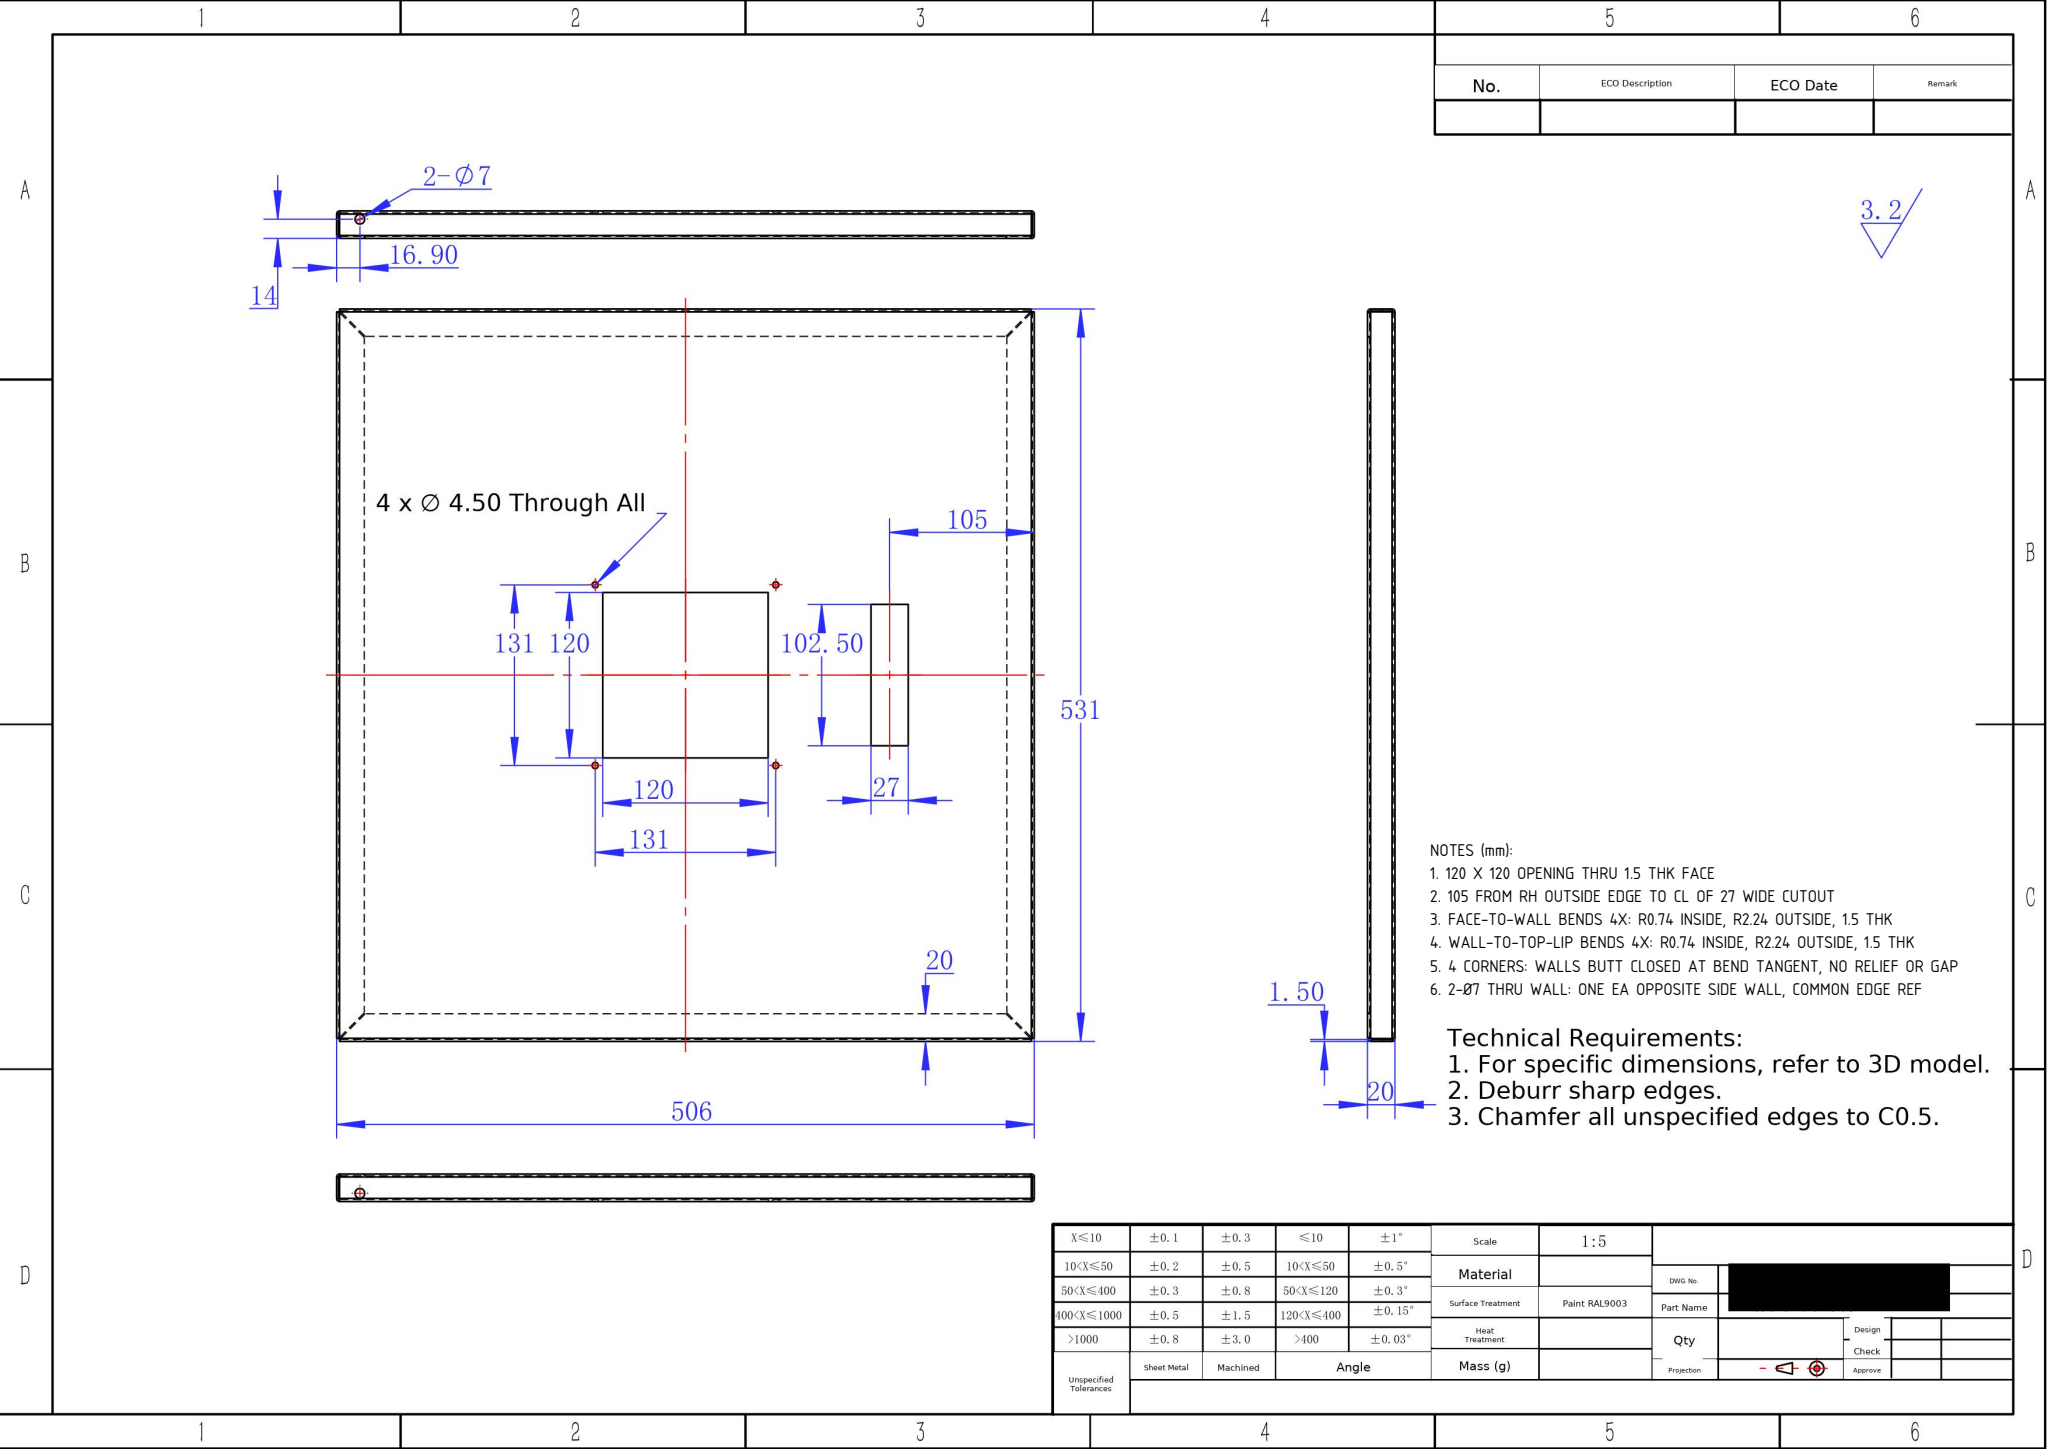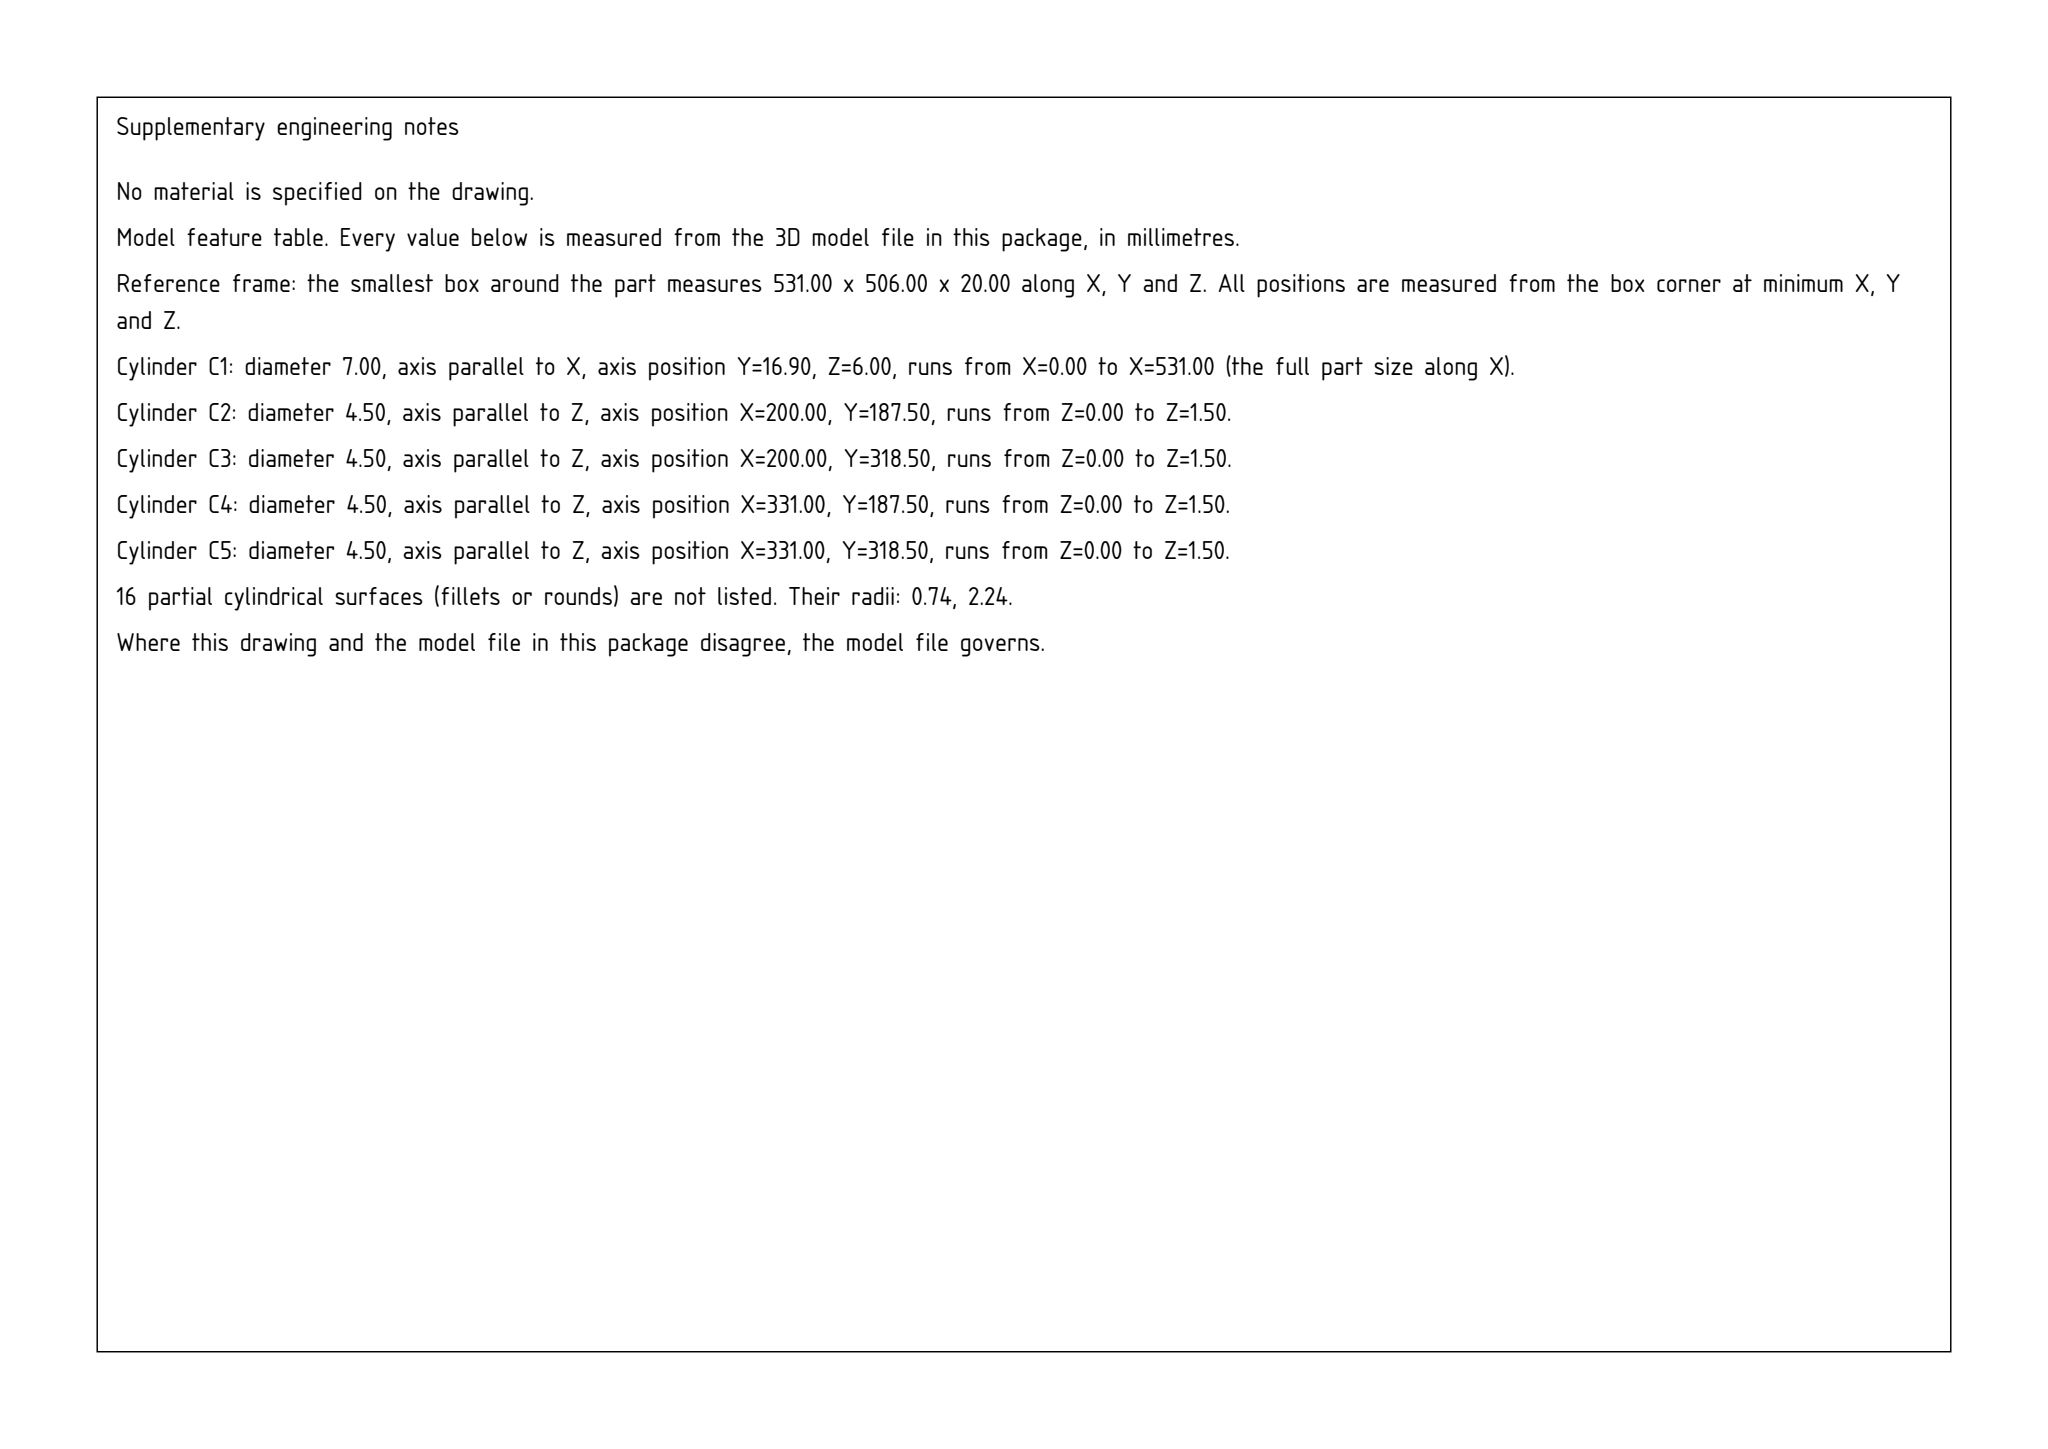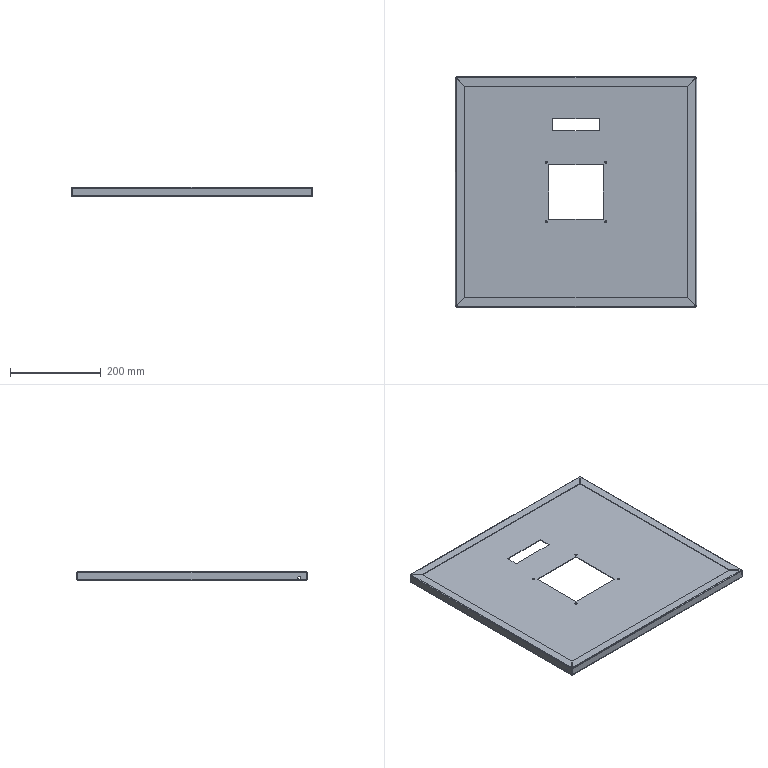Part | SolidWorks | mm | 1 solid | 90 faces | box 531 x 506 x 20 mm | volume 485168 mm3 | plane 46 | cylinder 28 | spline 16 | commonest cylinder face diameters 4.5 x8 4.473 x8 1.473 x8 7 x4
Drawing notes:
120 X 120 OPENING THRU 1.5 THK FACE | from the solid: opening x=205.52..325.52, y=193.02..313.02; face between z=0.02 and 1.52 = 1.5 thk
105 FROM RH OUTSIDE EDGE TO CL OF 27 WIDE CUTOUT | from the solid: cutout y=387.52..414.52 (27 wide), CL y=401.02; outer face y=506.02; 506.02-401.02=105.00
FACE-TO-WALL BENDS 4X: R0.74 INSIDE, R2.24 OUTSIDE, 1.5 THK | from the solid: Ø1.473 inner + Ø4.473 outer bend cylinders at 2.25 offsets on all 4 face/wall bends
WALL-TO-TOP-LIP BENDS 4X: R0.74 INSIDE, R2.24 OUTSIDE, 1.5 THK | from the solid: Ø1.473/Ø4.473 cyls axes at z=17.78 along X (y=2.25/503.78) and Y (x=2.25/528.78); z planes 18.52/20.02
4 CORNERS: WALLS BUTT CLOSED AT BEND TANGENT, NO RELIEF OR GAP | from the solid: X-bend cyl L=526.59 (x 2.22-528.81) meets Y-bend cyl L=501.59 (y 2.22-503.81)
2-Ø7 THRU WALL: ONE EA OPPOSITE SIDE WALL, COMMON EDGE REF | from the solid: Ø7.0 cyls, axis X, both y=16.92, z=6.02, L=1.5 = wall thk; walls x=0.02-1.52 and x=529.52-531.02